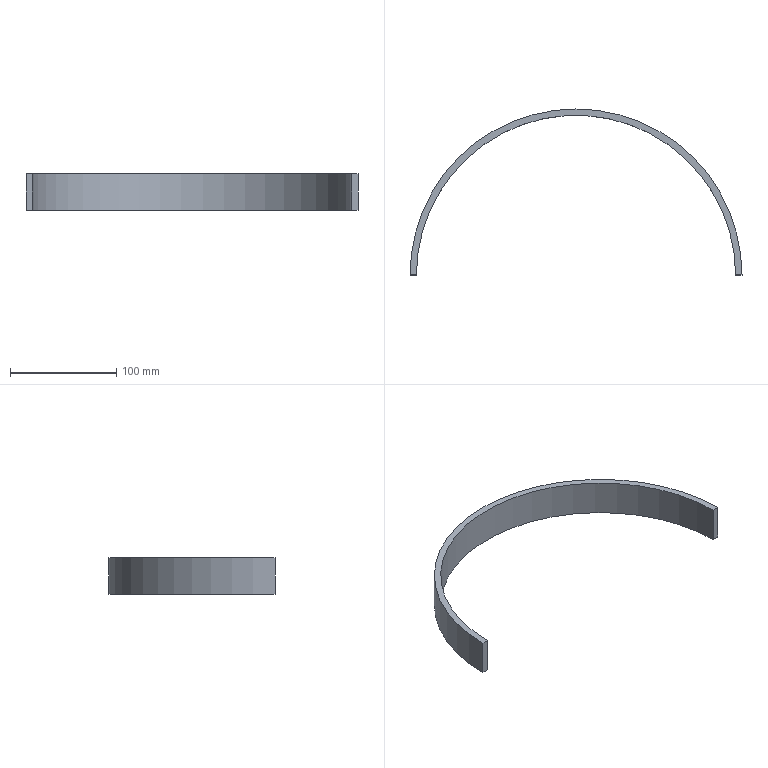Component | SolidWorks | JF21-80.1-1-3(_)-1-SOLID28-1 | 1 solid | 6 faces | box 312 x 156 x 34 mm | volume 98055 mm3 | plane 4 | cylinder 2 | commonest cylinder face diameters 300 x1 312 x1
STEP:
#1=COLOUR_RGB('',0.7922,0.8196,0.9333);
#2=FILL_AREA_STYLE_COLOUR('',#1);
#3=FILL_AREA_STYLE('',(#2));
#4=SURFACE_STYLE_FILL_AREA(#3);
#5=SURFACE_SIDE_STYLE('',(#4));
#6=SURFACE_STYLE_USAGE(.BOTH.,#5);
#7=PRESENTATION_STYLE_ASSIGNMENT((#6));
#8=CARTESIAN_POINT('',(5.906,-0.,11.22));
#9=VERTEX_POINT('',#8);
#10=CARTESIAN_POINT('',(-5.906,-0.,11.22));
#11=VERTEX_POINT('',#10);
#12=CARTESIAN_POINT('',(0.,0.,11.22));
#13=DIRECTION('',(0.,0.,1.));
#14=DIRECTION('',(1.,0.,0.));
#15=AXIS2_PLACEMENT_3D('',#12,#13,#14);
#16=CIRCLE('',#15,5.906);
#17=EDGE_CURVE('',#9,#11,#16,.T.);
#18=ORIENTED_EDGE('',*,*,#17,.T.);
#19=CARTESIAN_POINT('',(-6.142,-0.,11.22));
#20=VERTEX_POINT('',#19);
#21=CARTESIAN_POINT('',(-6.142,-0.,11.22));
#22=DIRECTION('',(-1.,-0.,0.));
#23=VECTOR('',#22,39.37);
#24=LINE('',#21,#23);
#25=EDGE_CURVE('',#11,#20,#24,.T.);
#26=ORIENTED_EDGE('',*,*,#25,.T.);
#27=CARTESIAN_POINT('',(6.142,-0.,11.22));
#28=VERTEX_POINT('',#27);
#29=CARTESIAN_POINT('',(0.,0.,11.22));
#30=DIRECTION('',(0.,0.,1.));
#31=DIRECTION('',(1.,0.,0.));
#32=AXIS2_PLACEMENT_3D('',#29,#30,#31);
#33=CIRCLE('',#32,6.142);
#34=EDGE_CURVE('',#28,#20,#33,.T.);
#35=ORIENTED_EDGE('',*,*,#34,.F.);
#36=CARTESIAN_POINT('',(6.142,-0.,11.22));
#37=DIRECTION('',(1.,-0.,0.));
#38=VECTOR('',#37,39.37);
#39=LINE('',#36,#38);
#40=EDGE_CURVE('',#9,#28,#39,.T.);
#41=ORIENTED_EDGE('',*,*,#40,.F.);
#42=EDGE_LOOP('',(#18,#26,#35,#41));
#43=FACE_OUTER_BOUND('',#42,.T.);
#44=CARTESIAN_POINT('',(6.142,-0.,11.22));
#45=DIRECTION('',(0.,0.,1.));
#46=DIRECTION('',(-1.,0.,0.));
#47=AXIS2_PLACEMENT_3D('',#44,#45,#46);
#48=PLANE('',#47);
#49=ADVANCED_FACE('',(#43),#48,.F.);
#50=CARTESIAN_POINT('',(5.906,-0.,12.559));
#51=VERTEX_POINT('',#50);
#52=CARTESIAN_POINT('',(-5.906,-0.,12.559));
#53=VERTEX_POINT('',#52);
#54=CARTESIAN_POINT('',(0.,0.,12.559));
#55=DIRECTION('',(0.,0.,1.));
#56=DIRECTION('',(1.,0.,0.));
#57=AXIS2_PLACEMENT_3D('',#54,#55,#56);
#58=CIRCLE('',#57,5.906);
#59=EDGE_CURVE('',#51,#53,#58,.T.);
#60=ORIENTED_EDGE('',*,*,#59,.T.);
#61=CARTESIAN_POINT('',(-5.906,-0.,11.22));
#62=DIRECTION('',(-0.,-0.,-1.));
#63=VECTOR('',#62,39.37);
#64=LINE('',#61,#63);
#65=EDGE_CURVE('',#53,#11,#64,.T.);
#66=ORIENTED_EDGE('',*,*,#65,.T.);
#67=ORIENTED_EDGE('',*,*,#17,.F.);
#68=CARTESIAN_POINT('',(5.906,-0.,11.22));
#69=DIRECTION('',(0.,-0.,-1.));
#70=VECTOR('',#69,39.37);
#71=LINE('',#68,#70);
#72=EDGE_CURVE('',#51,#9,#71,.T.);
#73=ORIENTED_EDGE('',*,*,#72,.F.);
#74=EDGE_LOOP('',(#60,#66,#67,#73));
#75=FACE_OUTER_BOUND('',#74,.T.);
#76=CARTESIAN_POINT('',(0.,0.,17.45));
#77=DIRECTION('',(0.,0.,1.));
#78=DIRECTION('',(-1.,0.,0.));
#79=AXIS2_PLACEMENT_3D('',#76,#77,#78);
#80=CYLINDRICAL_SURFACE('',#79,5.906);
#81=ADVANCED_FACE('',(#75),#80,.F.);
#82=CARTESIAN_POINT('',(6.142,-0.,12.559));
#83=VERTEX_POINT('',#82);
#84=CARTESIAN_POINT('',(-6.142,-0.,12.559));
#85=VERTEX_POINT('',#84);
#86=CARTESIAN_POINT('',(0.,0.,12.559));
#87=DIRECTION('',(0.,0.,1.));
#88=DIRECTION('',(1.,0.,0.));
#89=AXIS2_PLACEMENT_3D('',#86,#87,#88);
#90=CIRCLE('',#89,6.142);
#91=EDGE_CURVE('',#83,#85,#90,.T.);
#92=ORIENTED_EDGE('',*,*,#91,.T.);
#93=CARTESIAN_POINT('',(-5.906,-0.,12.559));
#94=DIRECTION('',(1.,0.,0.));
#95=VECTOR('',#94,39.37);
#96=LINE('',#93,#95);
#97=EDGE_CURVE('',#85,#53,#96,.T.);
#98=ORIENTED_EDGE('',*,*,#97,.T.);
#99=ORIENTED_EDGE('',*,*,#59,.F.);
#100=CARTESIAN_POINT('',(5.906,-0.,12.559));
#101=DIRECTION('',(-1.,0.,0.));
#102=VECTOR('',#101,39.37);
#103=LINE('',#100,#102);
#104=EDGE_CURVE('',#83,#51,#103,.T.);
#105=ORIENTED_EDGE('',*,*,#104,.F.);
#106=EDGE_LOOP('',(#92,#98,#99,#105));
#107=FACE_OUTER_BOUND('',#106,.T.);
#108=CARTESIAN_POINT('',(5.906,-0.,12.559));
#109=DIRECTION('',(0.,0.,-1.));
#110=DIRECTION('',(1.,0.,0.));
#111=AXIS2_PLACEMENT_3D('',#108,#109,#110);
#112=PLANE('',#111);
#113=ADVANCED_FACE('',(#107),#112,.F.);
#114=ORIENTED_EDGE('',*,*,#40,.T.);
#115=CARTESIAN_POINT('',(6.142,-0.,12.559));
#116=DIRECTION('',(0.,0.,1.));
#117=VECTOR('',#116,39.37);
#118=LINE('',#115,#117);
#119=EDGE_CURVE('',#28,#83,#118,.T.);
#120=ORIENTED_EDGE('',*,*,#119,.T.);
#121=ORIENTED_EDGE('',*,*,#104,.T.);
#122=ORIENTED_EDGE('',*,*,#72,.T.);
#123=EDGE_LOOP('',(#114,#120,#121,#122));
#124=FACE_OUTER_BOUND('',#123,.T.);
#125=CARTESIAN_POINT('',(5.906,-0.,11.22));
#126=DIRECTION('',(0.,1.,0.));
#127=DIRECTION('',(0.,0.,-1.));
#128=AXIS2_PLACEMENT_3D('',#125,#126,#127);
#129=PLANE('',#128);
#130=ADVANCED_FACE('',(#124),#129,.F.);
#131=ORIENTED_EDGE('',*,*,#119,.F.);
#132=ORIENTED_EDGE('',*,*,#34,.T.);
#133=CARTESIAN_POINT('',(-6.142,-0.,12.559));
#134=DIRECTION('',(0.,0.,1.));
#135=VECTOR('',#134,39.37);
#136=LINE('',#133,#135);
#137=EDGE_CURVE('',#20,#85,#136,.T.);
#138=ORIENTED_EDGE('',*,*,#137,.T.);
#139=ORIENTED_EDGE('',*,*,#91,.F.);
#140=EDGE_LOOP('',(#131,#132,#138,#139));
#141=FACE_OUTER_BOUND('',#140,.T.);
#142=CARTESIAN_POINT('',(0.,0.,17.45));
#143=DIRECTION('',(0.,0.,1.));
#144=DIRECTION('',(-1.,0.,0.));
#145=AXIS2_PLACEMENT_3D('',#142,#143,#144);
#146=CYLINDRICAL_SURFACE('',#145,6.142);
#147=ADVANCED_FACE('',(#141),#146,.T.);
#148=ORIENTED_EDGE('',*,*,#25,.F.);
#149=ORIENTED_EDGE('',*,*,#65,.F.);
#150=ORIENTED_EDGE('',*,*,#97,.F.);
#151=ORIENTED_EDGE('',*,*,#137,.F.);
#152=EDGE_LOOP('',(#148,#149,#150,#151));
#153=FACE_OUTER_BOUND('',#152,.T.);
#154=CARTESIAN_POINT('',(-5.906,-0.,11.22));
#155=DIRECTION('',(0.,-1.,0.));
#156=DIRECTION('',(0.,0.,-1.));
#157=AXIS2_PLACEMENT_3D('',#154,#155,#156);
#158=PLANE('',#157);
#159=ADVANCED_FACE('',(#153),#158,.T.);
#160=CLOSED_SHELL('',(#49,#81,#113,#130,#147,#159));
#161=MANIFOLD_SOLID_BREP('',#160);
#162=STYLED_ITEM('',(#7),#161);
#163=PRESENTATION_LAYER_ASSIGNMENT('','',(#162));
#164=CARTESIAN_POINT('',(0.,0.,0.));
#165=DIRECTION('',(0.,0.,1.));
#166=DIRECTION('',(1.,0.,0.));
#167=AXIS2_PLACEMENT_3D('',#164,#165,#166);
#168=(LENGTH_UNIT()NAMED_UNIT(*)SI_UNIT($,.METRE.));
#169=LENGTH_MEASURE_WITH_UNIT(LENGTH_MEASURE(0.0254),#168);
#170=DIMENSIONAL_EXPONENTS(1.,0.,0.,0.,0.,0.,0.);
#171=(CONVERSION_BASED_UNIT('',#169)LENGTH_UNIT()NAMED_UNIT(#170));
#172=UNCERTAINTY_MEASURE_WITH_UNIT(LENGTH_MEASURE(0.00001),#171,'','');
#173=(NAMED_UNIT(*)PLANE_ANGLE_UNIT()SI_UNIT($,.RADIAN.));
#174=(NAMED_UNIT(*)SI_UNIT($,.STERADIAN.)SOLID_ANGLE_UNIT());
#175=(GEOMETRIC_REPRESENTATION_CONTEXT(3)GLOBAL_UNCERTAINTY_ASSIGNED_CONTEXT((#172))GLOBAL_UNIT_ASSIGNED_CONTEXT((#171,#173,#174))REPRESENTATION_CONTEXT('',''));
#176=ADVANCED_BREP_SHAPE_REPRESENTATION('',(#161,#167),#175);
#177=(LENGTH_UNIT()NAMED_UNIT(*)SI_UNIT($,.METRE.));
#178=LENGTH_MEASURE_WITH_UNIT(LENGTH_MEASURE(0.0254),#177);
#179=DIMENSIONAL_EXPONENTS(1.,0.,0.,0.,0.,0.,0.);
#180=(CONVERSION_BASED_UNIT('',#178)LENGTH_UNIT()NAMED_UNIT(#179));
#181=UNCERTAINTY_MEASURE_WITH_UNIT(LENGTH_MEASURE(0.00001),#180,'','');
#182=(NAMED_UNIT(*)PLANE_ANGLE_UNIT()SI_UNIT($,.RADIAN.));
#183=(NAMED_UNIT(*)SI_UNIT($,.STERADIAN.)SOLID_ANGLE_UNIT());
#184=(GEOMETRIC_REPRESENTATION_CONTEXT(3)GLOBAL_UNCERTAINTY_ASSIGNED_CONTEXT((#181))GLOBAL_UNIT_ASSIGNED_CONTEXT((#180,#182,#183))REPRESENTATION_CONTEXT('',''));
#185=MECHANICAL_DESIGN_GEOMETRIC_PRESENTATION_REPRESENTATION('',(#162),#184);